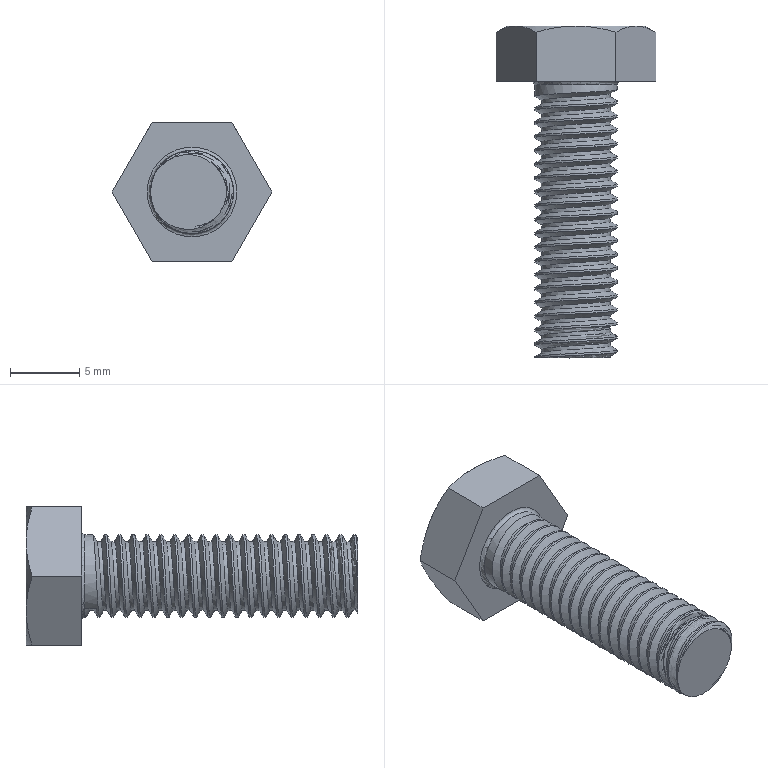Component | NX | M6X20_EXT | 1 solid | 21 faces | volume 816 mm3 | plane 10 | cone 6 | cylinder 2 | spline 2 | torus 1 | commonest cylinder face diameters 6 x1 5 x1